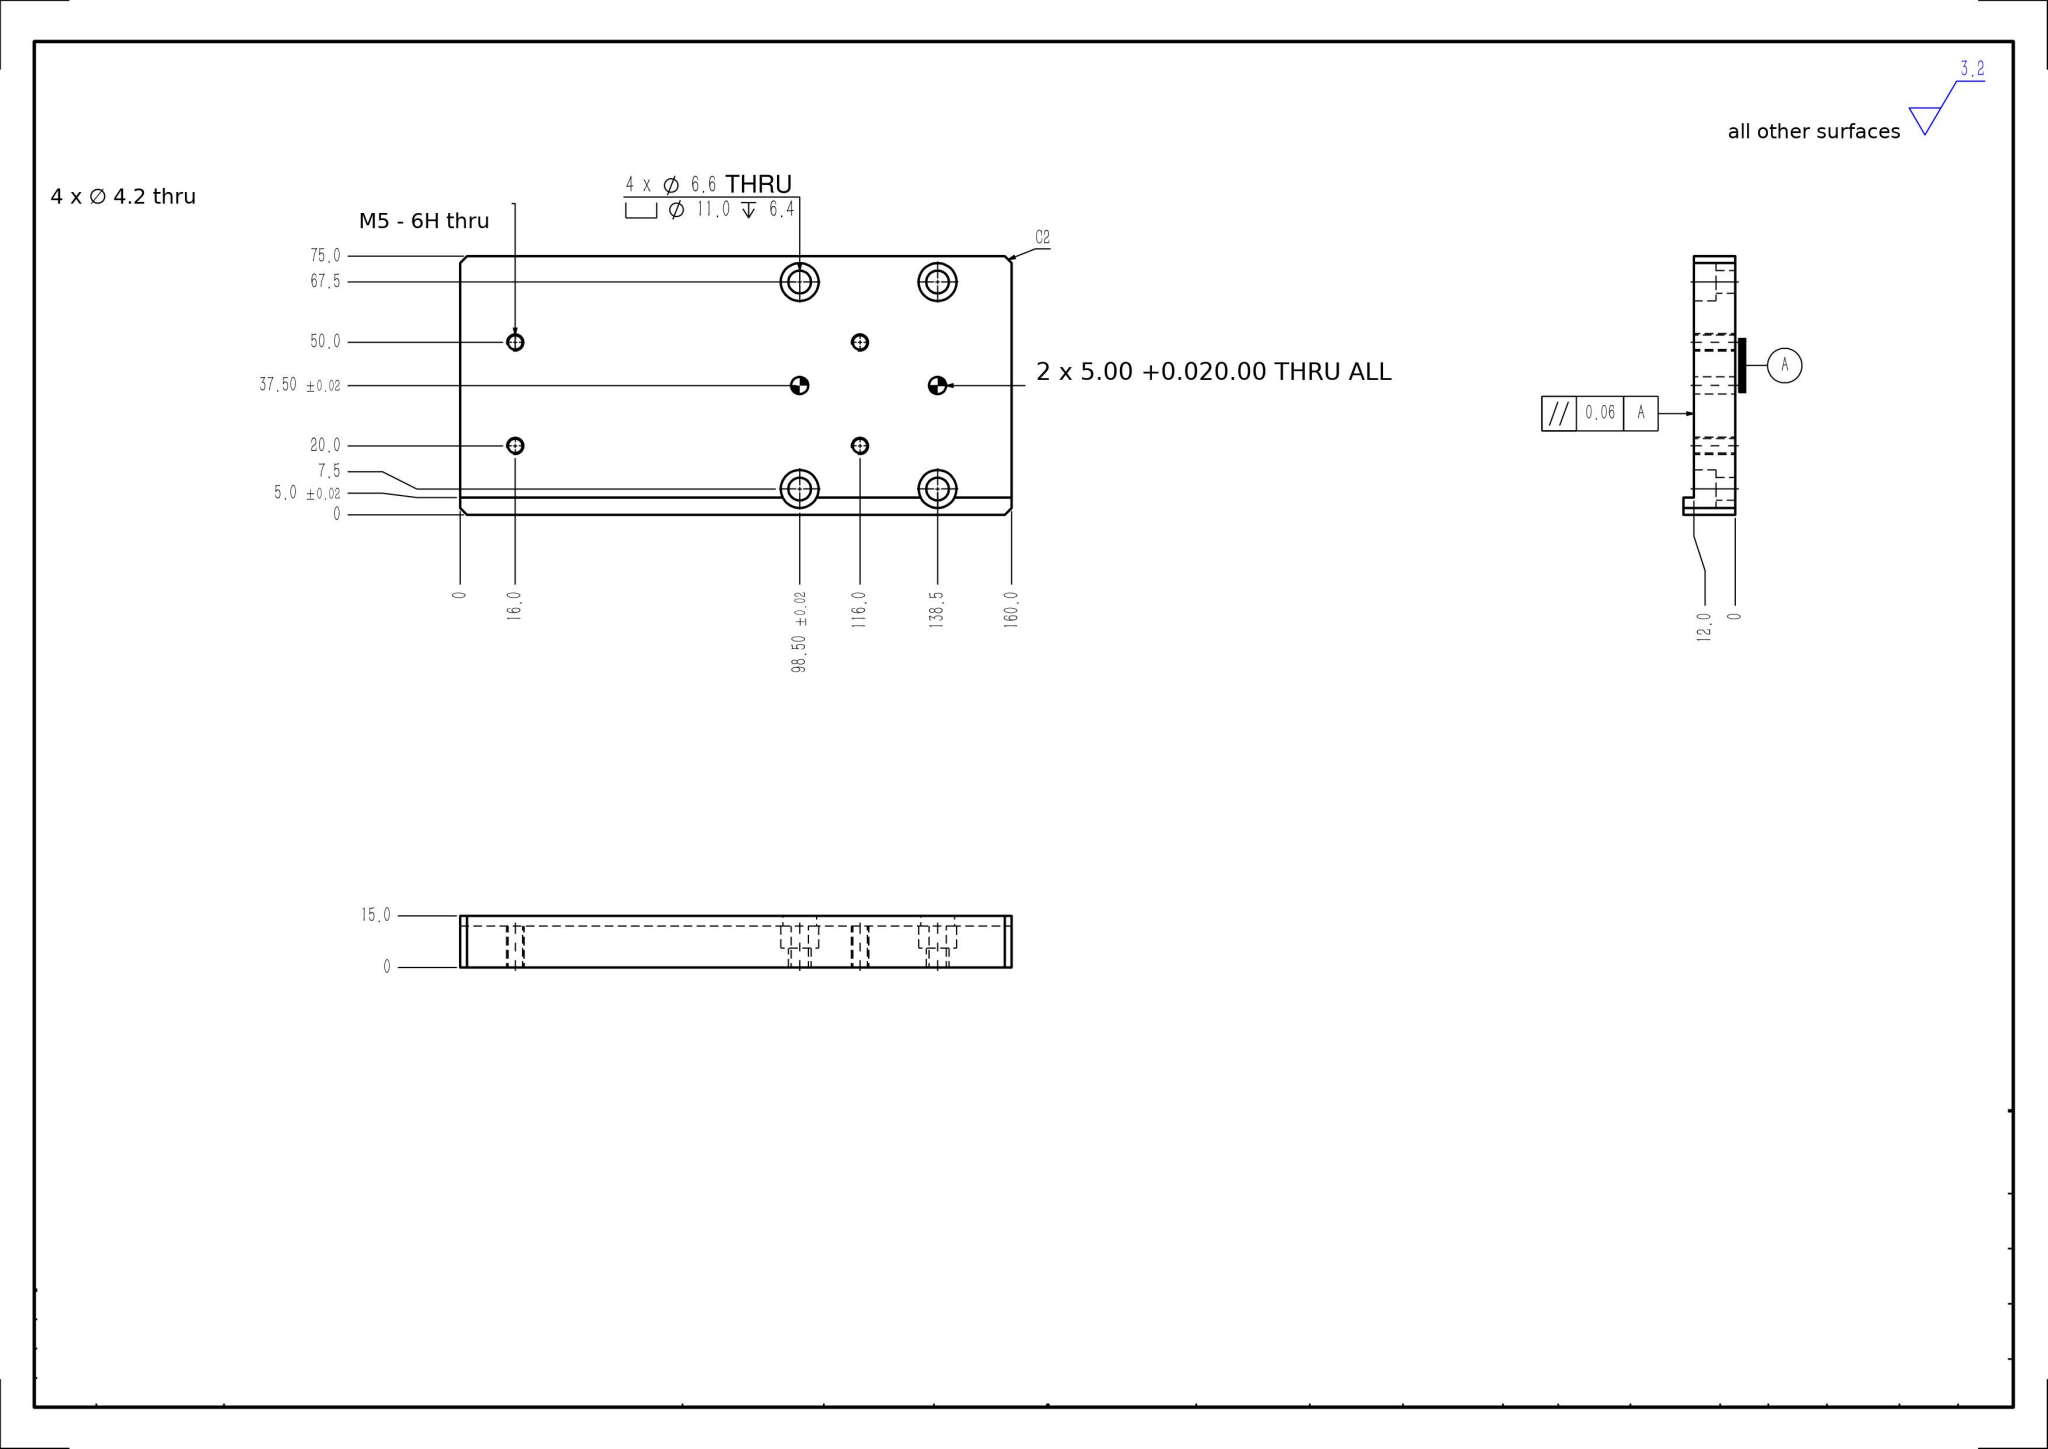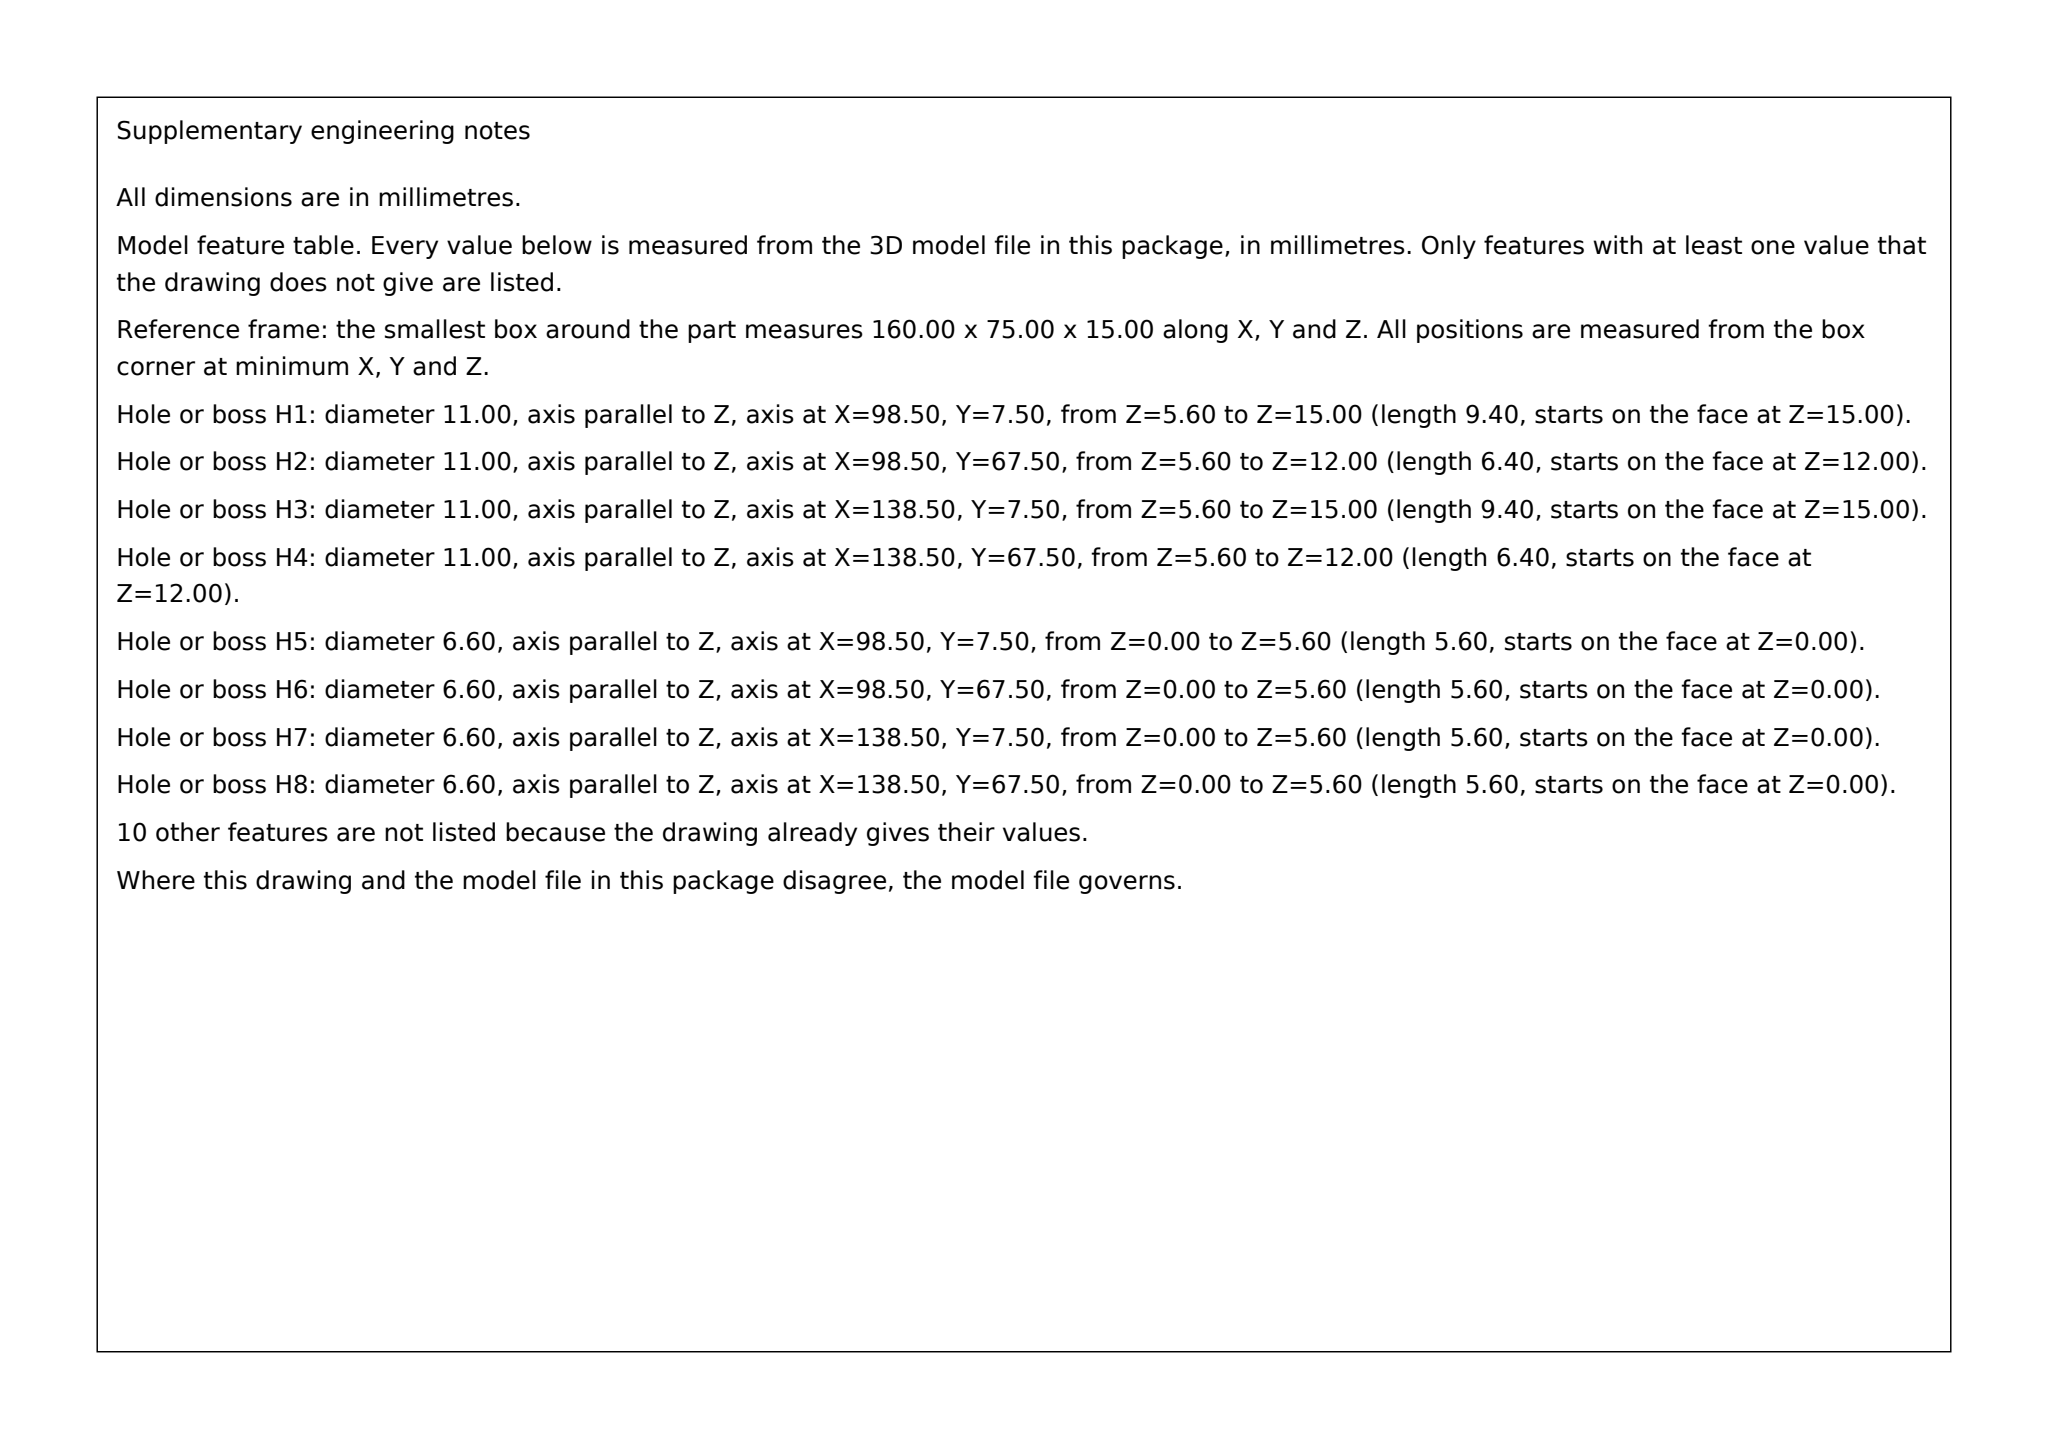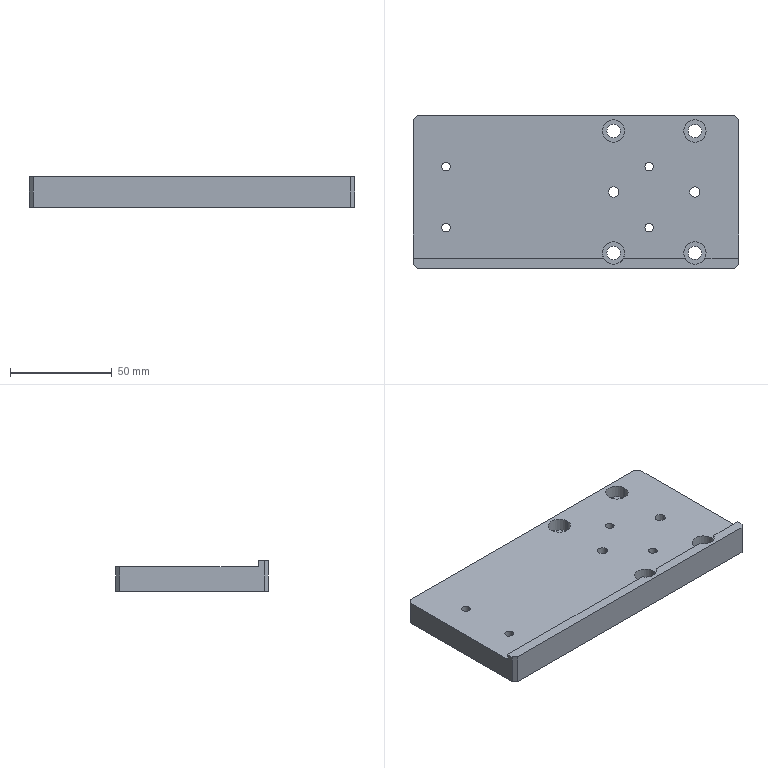Part | SolidWorks | mm | 1 solid | 46 faces | box 160 x 75 x 15 mm | volume 141831 mm3 | cylinder 28 | plane 18 | commonest cylinder face diameters 11 x8 6.6 x8 4.2 x8 5 x4
build123d program:
from build123d import *

# Parameters (mm, degrees)
SKETCH1_W                                      = 160
SKETCH1_H                                      = 75
BOSS_EXTRUDE1_DEPTH                            = 7.5
SKETCH2_W                                      = 160
SKETCH2_H                                      = 70
CUT_EXTRUDE1_DEPTH                             = 3
M5_TAPPED_HOLE1_D                              = 4.2
M6_HEX_SOCKET_HEAD_CAP_SCREW_CBORE1_AT_2_COUNT = 2
M6_HEX_SOCKET_HEAD_CAP_SCREW_CBORE1_AT_2_PITCH = 40
M6_HEX_SOCKET_HEAD_CAP_SCREW_CBORE1_AT_3_COUNT = 2
M6_HEX_SOCKET_HEAD_CAP_SCREW_CBORE1_AT_3_PITCH = 60
M6_HEX_SOCKET_HEAD_CAP_SCREW_CBORE1_AT_4_COUNT = 2
M6_HEX_SOCKET_HEAD_CAP_SCREW_CBORE1_AT_4_PITCH = 72.111
CUT_EXTRUDE2_START                             = 10
SKETCH7_R                                      = 5.5
CUT_EXTRUDE2_DEPTH                             = 10
SIZE_MM_DOWEL_PIN_HOLE1_D                      = 5
CHAMFER1_SIZE                                  = 2


with BuildPart() as part:
    # Sketch1 → Boss-Extrude1 (new, symmetric)
    with BuildSketch(Plane.XY):
        Rectangle(SKETCH1_W, SKETCH1_H)
    extrude(amount=BOSS_EXTRUDE1_DEPTH, both=True)

    # Sketch2 → Cut-Extrude1 (cut)
    with BuildSketch(Plane.XY.offset(7.5)):
        with Locations((0, 2.5)):
            Rectangle(SKETCH2_W, SKETCH2_H)
    extrude(amount=-CUT_EXTRUDE1_DEPTH, mode=Mode.SUBTRACT)

    # M5 Tapped Hole1 (through all)
    with Locations(Plane.XY.offset(4.5)):
        with Locations((36, 12.5), (36, -17.5), (-64, 12.5), (-64, -17.5)):
            Hole(M5_TAPPED_HOLE1_D / 2)

    # Sketch6 → M6 Hex Socket Head Cap Screw CBORE1 (revolve, cut)
    with BuildSketch(Plane(origin=(18.5, 30, 4.5), x_dir=(0, -1, 0), z_dir=(1, 0, 0))):
        Polygon((0, 0), (0, 12), (3.3, 12), (3.3, 6.4), (5.5, 6.4), (5.5, 0), align=None)
    m6_hex_socket_head_cap_screw_cbore1 = revolve(axis=Axis((18.5, 30, 10.85), (0, 0, -1)), mode=Mode.SUBTRACT)

    # M6 Hex Socket Head Cap Screw CBORE1 at 2: M6 Hex Socket Head Cap Screw CBORE1 ×2
    with Locations(*[(i * M6_HEX_SOCKET_HEAD_CAP_SCREW_CBORE1_AT_2_PITCH, 0, 0) for i in range(1, M6_HEX_SOCKET_HEAD_CAP_SCREW_CBORE1_AT_2_COUNT)]):
        add(m6_hex_socket_head_cap_screw_cbore1, mode=Mode.SUBTRACT)

    # M6 Hex Socket Head Cap Screw CBORE1 at 3: M6 Hex Socket Head Cap Screw CBORE1 ×2
    with Locations(*[(0, -i * M6_HEX_SOCKET_HEAD_CAP_SCREW_CBORE1_AT_3_PITCH, 0) for i in range(1, M6_HEX_SOCKET_HEAD_CAP_SCREW_CBORE1_AT_3_COUNT)]):
        add(m6_hex_socket_head_cap_screw_cbore1, mode=Mode.SUBTRACT)

    # M6 Hex Socket Head Cap Screw CBORE1 at 4: M6 Hex Socket Head Cap Screw CBORE1 ×2
    with Locations(*[Vector(0.5547, -0.8321, 0) * (i * M6_HEX_SOCKET_HEAD_CAP_SCREW_CBORE1_AT_4_PITCH) for i in range(1, M6_HEX_SOCKET_HEAD_CAP_SCREW_CBORE1_AT_4_COUNT)]):
        add(m6_hex_socket_head_cap_screw_cbore1, mode=Mode.SUBTRACT)

    # Sketch7 → Cut-Extrude2 (cut)
    with BuildSketch(Plane.XY.offset(-1.9).offset(CUT_EXTRUDE2_START)):
        with Locations((18.5, -30)):
            Circle(SKETCH7_R)
        with Locations((58.5, -30)):
            Circle(SKETCH7_R)
    extrude(amount=-CUT_EXTRUDE2_DEPTH, mode=Mode.SUBTRACT)

    # Size mm Dowel Pin Hole1 (through all)
    with Locations(Plane.XY.offset(4.5)):
        with Locations((18.5, 0), (58.5, 0)):
            Hole(SIZE_MM_DOWEL_PIN_HOLE1_D / 2)

    # Chamfer1
    chamfer1_edges = [part.edges().sort_by_distance(p)[0] for p in [
        (-80, 37.5, -1.5),
        (80, 37.5, -1.5),
        (80, -37.5, 0),
        (-80, -37.5, 0),
    ]]
    chamfer(chamfer1_edges, length=CHAMFER1_SIZE)


solid = part.part